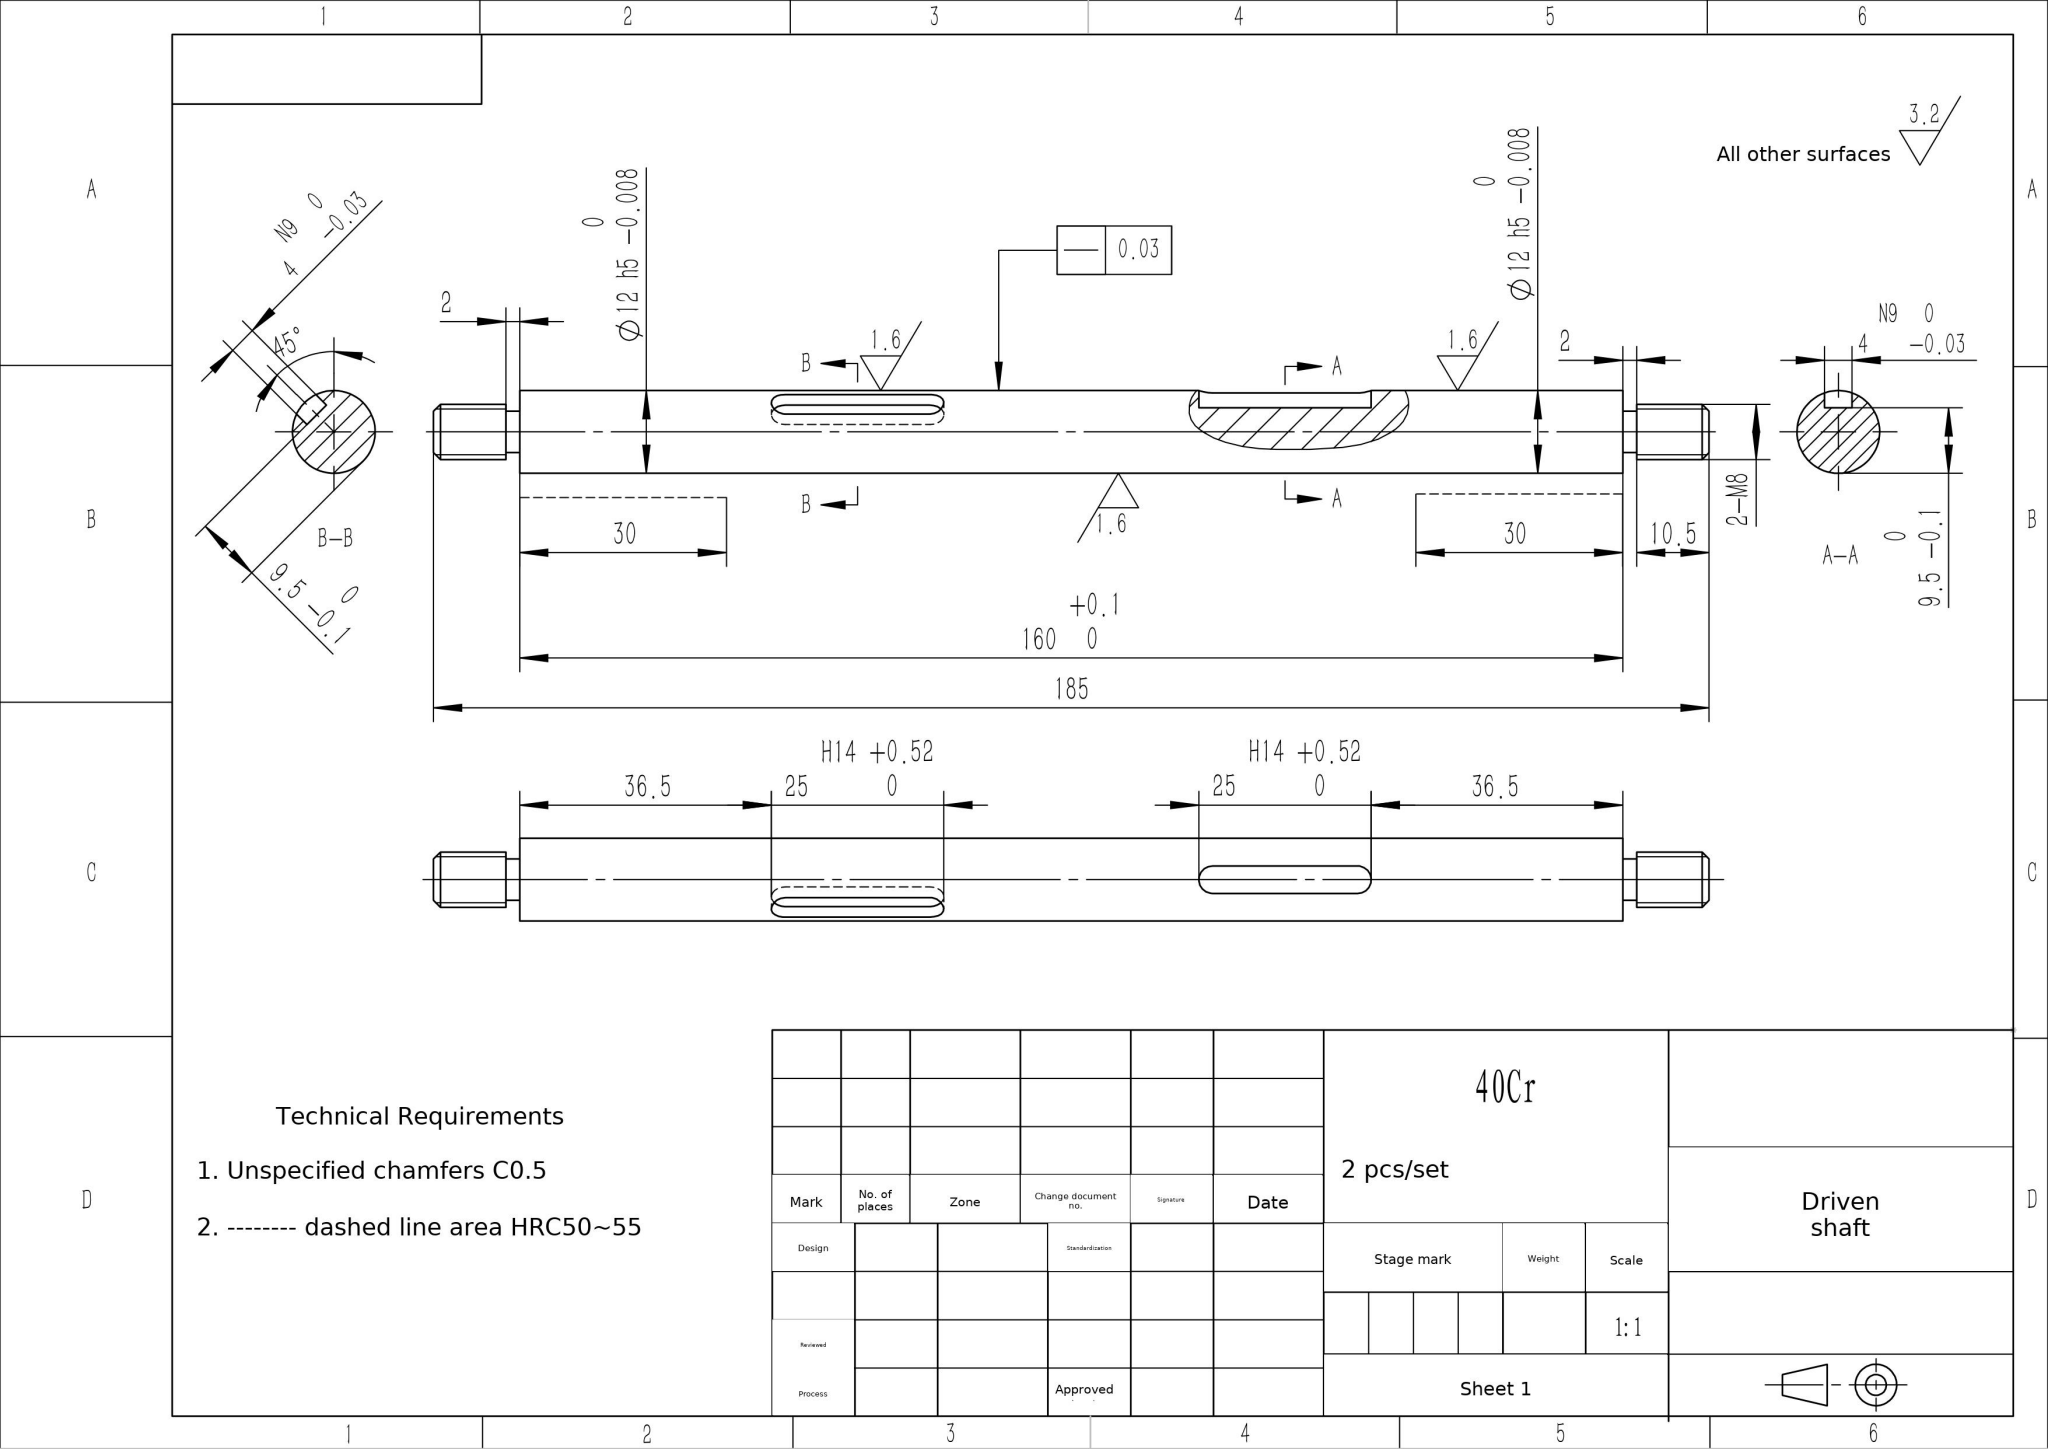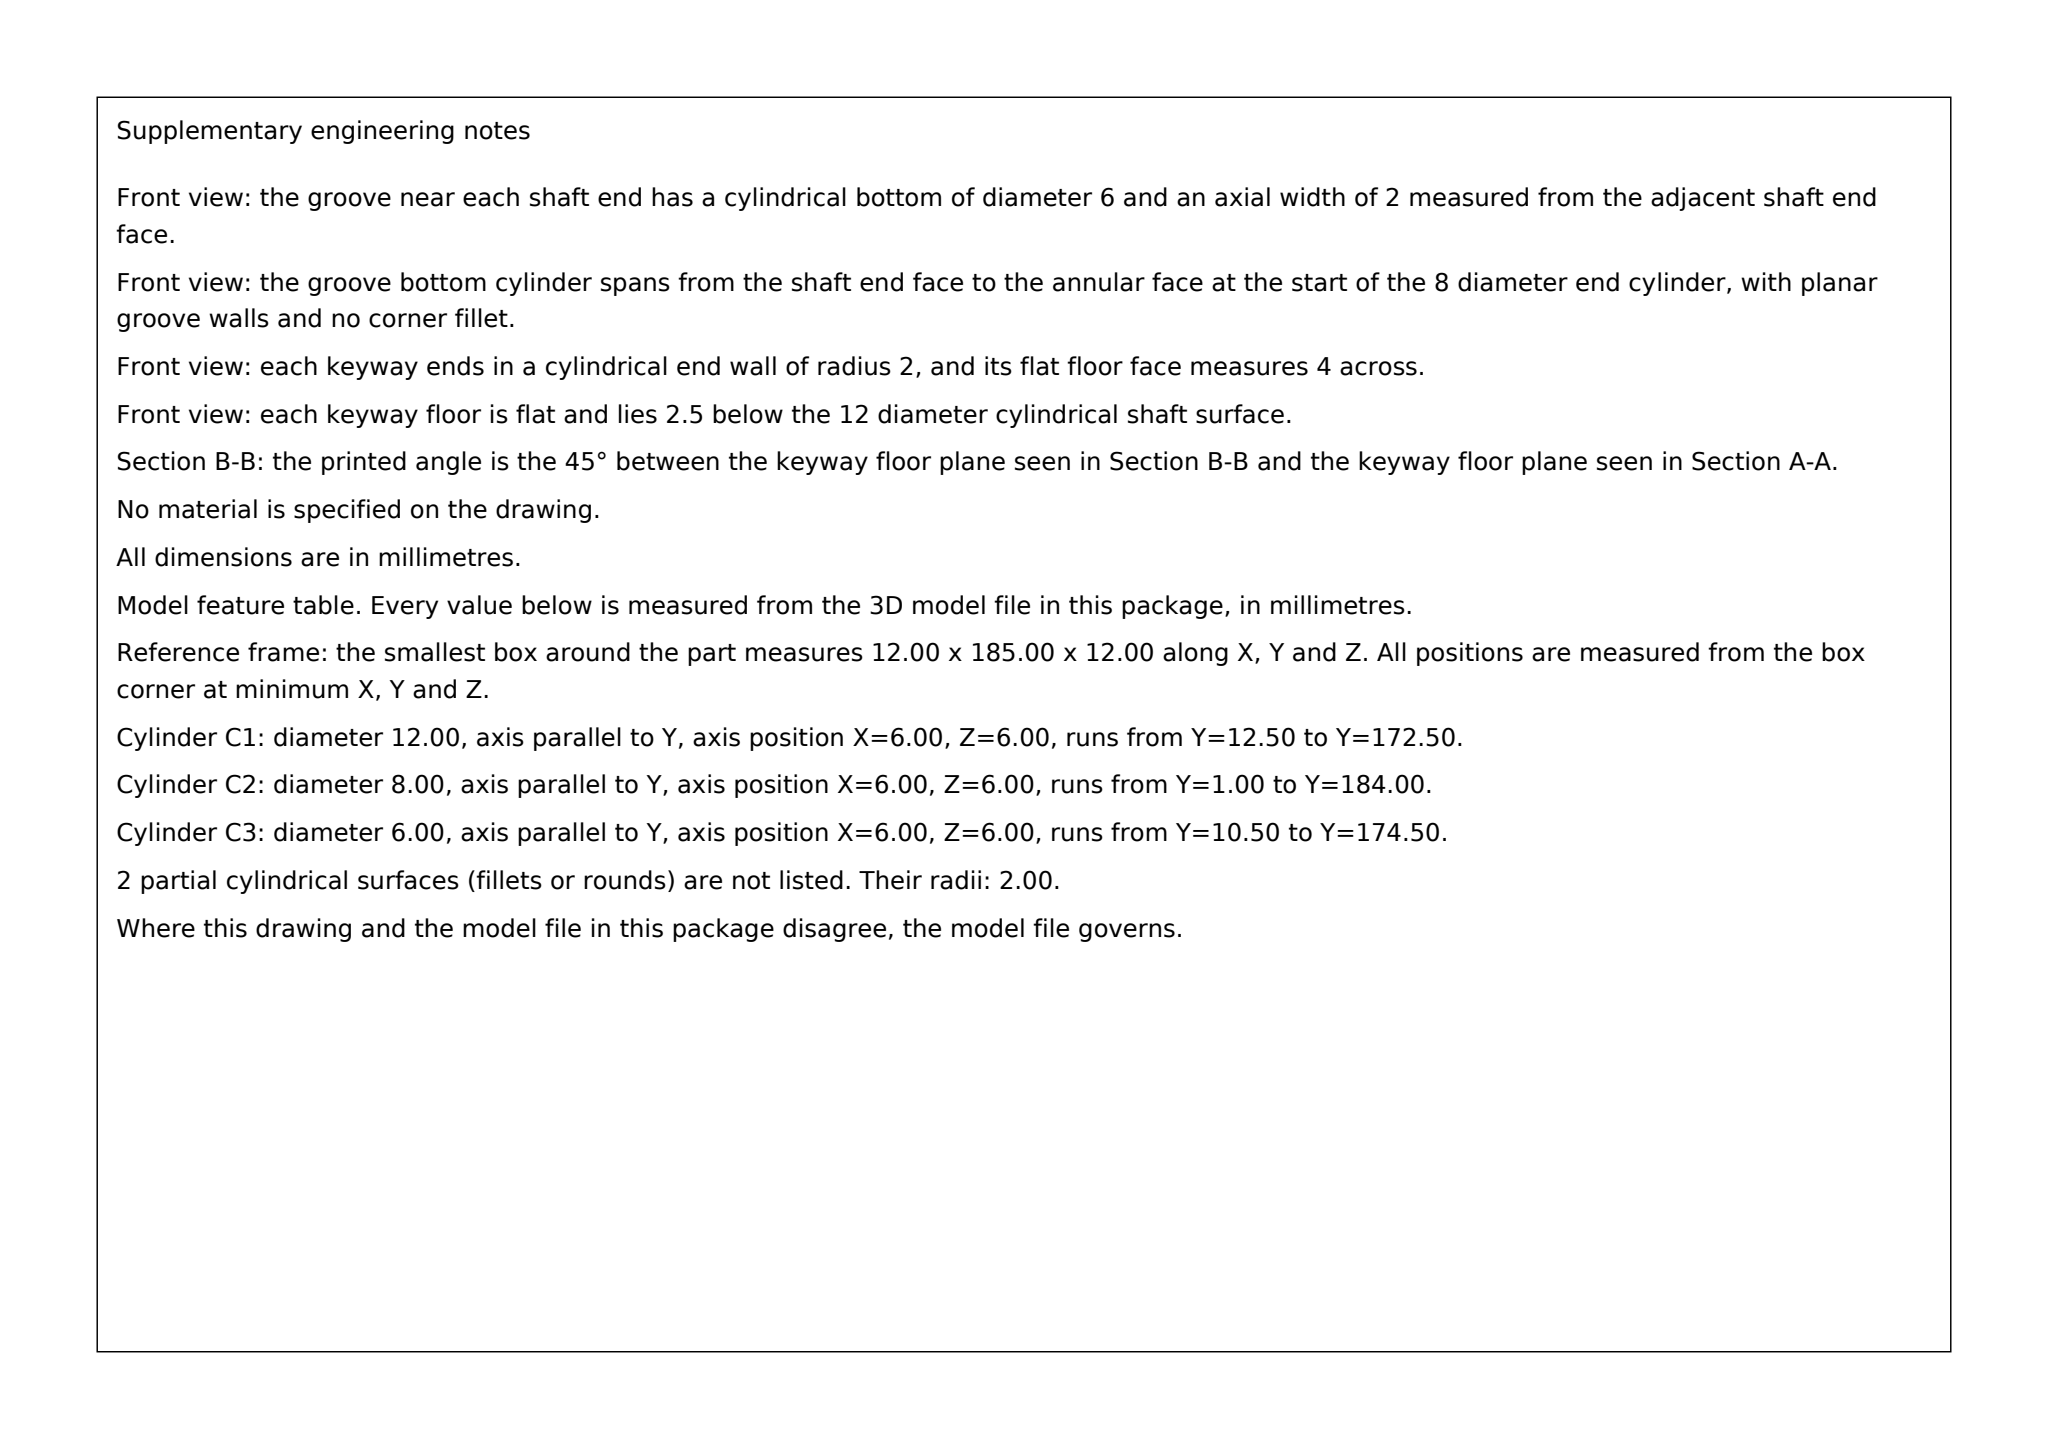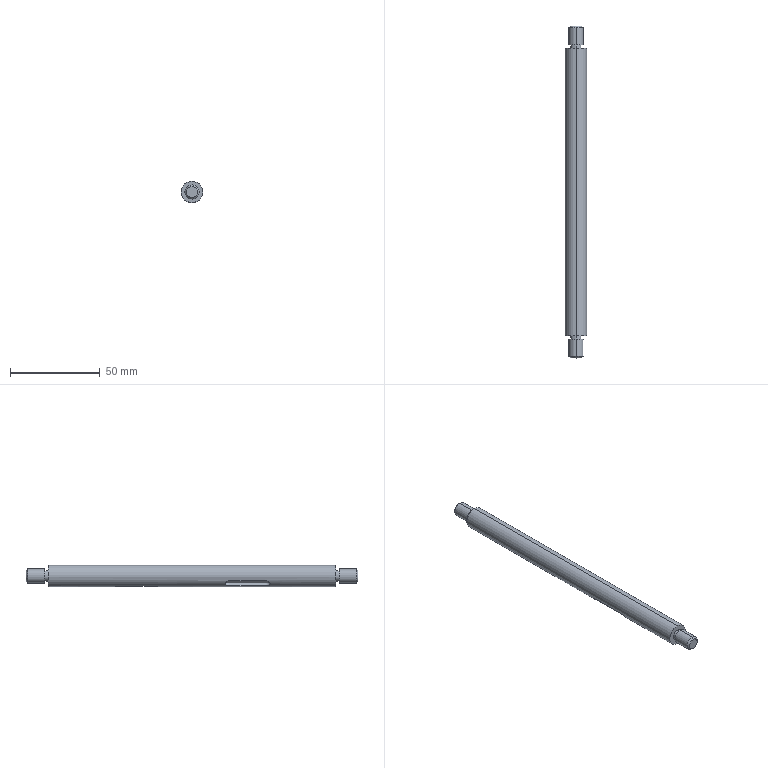Part | SolidWorks | mm | 1 solid | 30 faces | box 12 x 185 x 12 mm | volume 18779 mm3 | cylinder 14 | plane 12 | cone 4 | commonest cylinder face diameters 8 x4 6 x4 4 x4 12 x2
build123d program:
from build123d import *

# Parameters (mm, degrees)
SKETCH1_R           = 6
BOSS_EXTRUDE1_DEPTH = 92.5
CUT_EXTRUDE1_DEPTH  = 2.5
CUT_EXTRUDE2_DEPTH  = 2.5
SKETCH4_W           = 2
SKETCH4_H           = 12.5
CHAMFER2_SIZE       = 1
SKETCH5_W           = 1
SKETCH5_H           = 2


with BuildPart() as part:
    # Sketch1 → Boss-Extrude1 (new, symmetric)
    with BuildSketch(Plane(origin=(0, 0, 0), x_dir=(1, 0, 0), z_dir=(0, 1, 0))):
        with Locations(Location((0, 0, 0), (0, 0, 270))):
            Circle(SKETCH1_R)
    extrude(amount=BOSS_EXTRUDE1_DEPTH, both=True)

    # Sketch2 → Cut-Extrude1 (cut)
    with BuildSketch(Plane.XY.offset(-6)):
        with BuildLine():
            Line((2, 41.5), (2, 20.5))
            ThreePointArc((2, 20.5), (0, 18.5), (-2, 20.5))
            Line((-2, 20.5), (-2, 41.5))
            ThreePointArc((-2, 41.5), (0, 43.5), (2, 41.5))
        make_face()
    extrude(amount=CUT_EXTRUDE1_DEPTH, mode=Mode.SUBTRACT)

    # Sketch3 → Cut-Extrude2 (cut)
    with BuildSketch(Plane(origin=(-4.243, 0, -4.243), x_dir=(0, -1, 0), z_dir=(0.7071, 0, 0.7071))):
        with BuildLine():
            Line((20.5, 2), (41.5, 2))
            ThreePointArc((41.5, 2), (43.5, 0), (41.5, -2))
            Line((41.5, -2), (20.5, -2))
            ThreePointArc((20.5, -2), (18.5, 0), (20.5, 2))
        make_face()
    extrude(amount=CUT_EXTRUDE2_DEPTH, mode=Mode.SUBTRACT)

    # Sketch4 → Cut-Revolve3 (revolve, cut)
    with BuildSketch(Plane(origin=(0, 0, 0), x_dir=(0, 0, -1), z_dir=(1, 0, 0)), mode=Mode.PRIVATE) as cut_revolve3_sk:
        with Locations((-5, 86.25)):
            Rectangle(SKETCH4_W, SKETCH4_H)
        with Locations((-5, -86.25)):
            Rectangle(SKETCH4_W, SKETCH4_H)
    revolve(cut_revolve3_sk.sketch.rotate(Axis((0, -157.172, 0), (0, 1, 0)), 180), axis=Axis((0, -157.172, 0), (0, 1, 0)), mode=Mode.SUBTRACT)

    # Chamfer2
    chamfer2_edges = [part.edges().sort_by_distance(p)[0] for p in [
        (0, 92.5, 4),
        (0, -92.5, 4),
    ]]
    chamfer(chamfer2_edges, length=CHAMFER2_SIZE)

    # Sketch5 → Cut-Revolve4 (revolve, cut)
    with BuildSketch(Plane(origin=(0, 0, 0), x_dir=(0, 0, -1), z_dir=(1, 0, 0)), mode=Mode.PRIVATE) as cut_revolve4_sk:
        with Locations((-3.5, 81)):
            Rectangle(SKETCH5_W, SKETCH5_H)
    cut_revolve4 = revolve(cut_revolve4_sk.sketch.rotate(Axis((0, -119.118, 0), (0, 1, 0)), 180), axis=Axis((0, -119.118, 0), (0, 1, 0)), mode=Mode.SUBTRACT)

    # Mirror1: Cut-Revolve4 across plane
    add(cut_revolve4.mirror(Plane.ZX), mode=Mode.SUBTRACT)


solid = part.part